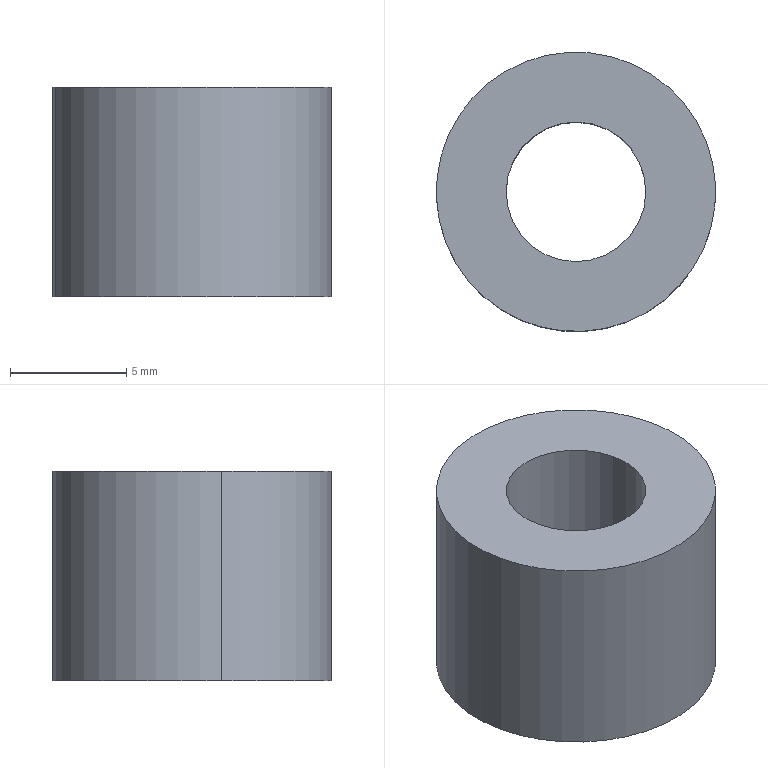Component | SolidWorks | ControlSleeve-1 | 1 solid | 6 faces | box 12 x 12 x 9 mm | volume 763 mm3 | cylinder 4 | plane 2 | commonest cylinder face diameters 6 x2 12 x2
build123d program:
from build123d import *

# Parameters (mm, degrees)
SKETCH1_R           = 6
SKETCH1_R_2         = 3
BOSS_EXTRUDE1_DEPTH = 9


with BuildPart() as part:
    # Sketch1 → Boss-Extrude1 (new body)
    with BuildSketch(Plane.XY):
        Circle(SKETCH1_R)
        Circle(SKETCH1_R_2, mode=Mode.SUBTRACT)
    extrude(amount=BOSS_EXTRUDE1_DEPTH)


solid = part.part

# Placed as in the assembly
solid = solid.moved(Location((3.727, 9.876, 358.846), (0, 0, 0)))
STEP:
#1=COLOUR_RGB('',0.7922,0.8196,0.9333);
#2=FILL_AREA_STYLE_COLOUR('',#1);
#3=FILL_AREA_STYLE('',(#2));
#4=SURFACE_STYLE_FILL_AREA(#3);
#5=SURFACE_SIDE_STYLE('',(#4));
#6=SURFACE_STYLE_USAGE(.BOTH.,#5);
#7=PRESENTATION_STYLE_ASSIGNMENT((#6));
#8=CARTESIAN_POINT('',(0.03129,0.3639,14.482));
#9=VERTEX_POINT('',#8);
#10=CARTESIAN_POINT('',(0.2622,0.4137,14.482));
#11=VERTEX_POINT('',#10);
#12=CARTESIAN_POINT('',(0.1467,0.3888,14.482));
#13=DIRECTION('',(0.,0.,1.));
#14=DIRECTION('',(0.9775,0.2111,0.));
#15=AXIS2_PLACEMENT_3D('',#12,#13,#14);
#16=CIRCLE('',#15,0.1181);
#17=EDGE_CURVE('',#9,#11,#16,.T.);
#18=ORIENTED_EDGE('',*,*,#17,.T.);
#19=CARTESIAN_POINT('',(0.2622,0.4137,14.128));
#20=VERTEX_POINT('',#19);
#21=CARTESIAN_POINT('',(0.2622,0.4137,14.482));
#22=DIRECTION('',(0.,0.,-1.));
#23=VECTOR('',#22,39.37);
#24=LINE('',#21,#23);
#25=EDGE_CURVE('',#11,#20,#24,.T.);
#26=ORIENTED_EDGE('',*,*,#25,.T.);
#27=CARTESIAN_POINT('',(0.03129,0.3639,14.128));
#28=VERTEX_POINT('',#27);
#29=CARTESIAN_POINT('',(0.1467,0.3888,14.128));
#30=DIRECTION('',(0.,0.,1.));
#31=DIRECTION('',(0.9775,0.2111,0.));
#32=AXIS2_PLACEMENT_3D('',#29,#30,#31);
#33=CIRCLE('',#32,0.1181);
#34=EDGE_CURVE('',#28,#20,#33,.T.);
#35=ORIENTED_EDGE('',*,*,#34,.F.);
#36=CARTESIAN_POINT('',(0.03129,0.3639,14.482));
#37=DIRECTION('',(0.,0.,-1.));
#38=VECTOR('',#37,39.37);
#39=LINE('',#36,#38);
#40=EDGE_CURVE('',#9,#28,#39,.T.);
#41=ORIENTED_EDGE('',*,*,#40,.F.);
#42=EDGE_LOOP('',(#18,#26,#35,#41));
#43=FACE_OUTER_BOUND('',#42,.T.);
#44=CARTESIAN_POINT('',(0.1467,0.3888,14.482));
#45=DIRECTION('',(0.,0.,-1.));
#46=DIRECTION('',(-0.9775,-0.2111,0.));
#47=AXIS2_PLACEMENT_3D('',#44,#45,#46);
#48=CYLINDRICAL_SURFACE('',#47,0.1181);
#49=ADVANCED_FACE('',(#43),#48,.F.);
#50=CARTESIAN_POINT('',(0.3776,0.4387,14.482));
#51=VERTEX_POINT('',#50);
#52=CARTESIAN_POINT('',(-0.08416,0.3389,14.482));
#53=VERTEX_POINT('',#52);
#54=CARTESIAN_POINT('',(0.1467,0.3888,14.482));
#55=DIRECTION('',(0.,0.,1.));
#56=DIRECTION('',(0.9775,0.2111,0.));
#57=AXIS2_PLACEMENT_3D('',#54,#55,#56);
#58=CIRCLE('',#57,0.2362);
#59=EDGE_CURVE('',#51,#53,#58,.T.);
#60=ORIENTED_EDGE('',*,*,#59,.F.);
#61=CARTESIAN_POINT('',(0.3776,0.4387,14.128));
#62=VERTEX_POINT('',#61);
#63=CARTESIAN_POINT('',(0.3776,0.4387,14.482));
#64=DIRECTION('',(0.,0.,-1.));
#65=VECTOR('',#64,39.37);
#66=LINE('',#63,#65);
#67=EDGE_CURVE('',#51,#62,#66,.T.);
#68=ORIENTED_EDGE('',*,*,#67,.T.);
#69=CARTESIAN_POINT('',(-0.08416,0.3389,14.128));
#70=VERTEX_POINT('',#69);
#71=CARTESIAN_POINT('',(0.1467,0.3888,14.128));
#72=DIRECTION('',(0.,0.,1.));
#73=DIRECTION('',(0.9775,0.2111,0.));
#74=AXIS2_PLACEMENT_3D('',#71,#72,#73);
#75=CIRCLE('',#74,0.2362);
#76=EDGE_CURVE('',#62,#70,#75,.T.);
#77=ORIENTED_EDGE('',*,*,#76,.T.);
#78=CARTESIAN_POINT('',(-0.08416,0.3389,14.482));
#79=DIRECTION('',(0.,0.,-1.));
#80=VECTOR('',#79,39.37);
#81=LINE('',#78,#80);
#82=EDGE_CURVE('',#53,#70,#81,.T.);
#83=ORIENTED_EDGE('',*,*,#82,.F.);
#84=EDGE_LOOP('',(#60,#68,#77,#83));
#85=FACE_OUTER_BOUND('',#84,.T.);
#86=CARTESIAN_POINT('',(0.1467,0.3888,14.482));
#87=DIRECTION('',(0.,0.,-1.));
#88=DIRECTION('',(-0.9775,-0.2111,0.));
#89=AXIS2_PLACEMENT_3D('',#86,#87,#88);
#90=CYLINDRICAL_SURFACE('',#89,0.2362);
#91=ADVANCED_FACE('',(#85),#90,.T.);
#92=CARTESIAN_POINT('',(0.1467,0.3888,14.482));
#93=DIRECTION('',(0.,0.,1.));
#94=DIRECTION('',(0.9775,0.2111,0.));
#95=AXIS2_PLACEMENT_3D('',#92,#93,#94);
#96=CIRCLE('',#95,0.2362);
#97=EDGE_CURVE('',#53,#51,#96,.T.);
#98=ORIENTED_EDGE('',*,*,#97,.T.);
#99=ORIENTED_EDGE('',*,*,#59,.T.);
#100=EDGE_LOOP('',(#98,#99));
#101=FACE_OUTER_BOUND('',#100,.T.);
#102=ORIENTED_EDGE('',*,*,#17,.F.);
#103=CARTESIAN_POINT('',(0.1467,0.3888,14.482));
#104=DIRECTION('',(0.,0.,1.));
#105=DIRECTION('',(0.9775,0.2111,0.));
#106=AXIS2_PLACEMENT_3D('',#103,#104,#105);
#107=CIRCLE('',#106,0.1181);
#108=EDGE_CURVE('',#11,#9,#107,.T.);
#109=ORIENTED_EDGE('',*,*,#108,.F.);
#110=EDGE_LOOP('',(#102,#109));
#111=FACE_BOUND('',#110,.T.);
#112=CARTESIAN_POINT('',(0.1467,0.3888,14.482));
#113=DIRECTION('',(0.,0.,1.));
#114=DIRECTION('',(0.9775,0.2111,0.));
#115=AXIS2_PLACEMENT_3D('',#112,#113,#114);
#116=PLANE('',#115);
#117=ADVANCED_FACE('',(#101,#111),#116,.T.);
#118=CARTESIAN_POINT('',(0.1467,0.3888,14.128));
#119=DIRECTION('',(0.,0.,1.));
#120=DIRECTION('',(0.9775,0.2111,0.));
#121=AXIS2_PLACEMENT_3D('',#118,#119,#120);
#122=CIRCLE('',#121,0.2362);
#123=EDGE_CURVE('',#70,#62,#122,.T.);
#124=ORIENTED_EDGE('',*,*,#123,.F.);
#125=ORIENTED_EDGE('',*,*,#76,.F.);
#126=EDGE_LOOP('',(#124,#125));
#127=FACE_OUTER_BOUND('',#126,.T.);
#128=ORIENTED_EDGE('',*,*,#34,.T.);
#129=CARTESIAN_POINT('',(0.1467,0.3888,14.128));
#130=DIRECTION('',(0.,0.,1.));
#131=DIRECTION('',(0.9775,0.2111,0.));
#132=AXIS2_PLACEMENT_3D('',#129,#130,#131);
#133=CIRCLE('',#132,0.1181);
#134=EDGE_CURVE('',#20,#28,#133,.T.);
#135=ORIENTED_EDGE('',*,*,#134,.T.);
#136=EDGE_LOOP('',(#128,#135));
#137=FACE_BOUND('',#136,.T.);
#138=CARTESIAN_POINT('',(0.1467,0.3888,14.128));
#139=DIRECTION('',(0.,0.,1.));
#140=DIRECTION('',(0.9775,0.2111,0.));
#141=AXIS2_PLACEMENT_3D('',#138,#139,#140);
#142=PLANE('',#141);
#143=ADVANCED_FACE('',(#127,#137),#142,.F.);
#144=ORIENTED_EDGE('',*,*,#67,.F.);
#145=ORIENTED_EDGE('',*,*,#97,.F.);
#146=ORIENTED_EDGE('',*,*,#82,.T.);
#147=ORIENTED_EDGE('',*,*,#123,.T.);
#148=EDGE_LOOP('',(#144,#145,#146,#147));
#149=FACE_OUTER_BOUND('',#148,.T.);
#150=CARTESIAN_POINT('',(0.1467,0.3888,14.482));
#151=DIRECTION('',(0.,0.,-1.));
#152=DIRECTION('',(-0.9775,-0.2111,0.));
#153=AXIS2_PLACEMENT_3D('',#150,#151,#152);
#154=CYLINDRICAL_SURFACE('',#153,0.2362);
#155=ADVANCED_FACE('',(#149),#154,.T.);
#156=ORIENTED_EDGE('',*,*,#25,.F.);
#157=ORIENTED_EDGE('',*,*,#108,.T.);
#158=ORIENTED_EDGE('',*,*,#40,.T.);
#159=ORIENTED_EDGE('',*,*,#134,.F.);
#160=EDGE_LOOP('',(#156,#157,#158,#159));
#161=FACE_OUTER_BOUND('',#160,.T.);
#162=CARTESIAN_POINT('',(0.1467,0.3888,14.482));
#163=DIRECTION('',(0.,0.,-1.));
#164=DIRECTION('',(-0.9775,-0.2111,0.));
#165=AXIS2_PLACEMENT_3D('',#162,#163,#164);
#166=CYLINDRICAL_SURFACE('',#165,0.1181);
#167=ADVANCED_FACE('',(#161),#166,.F.);
#168=CLOSED_SHELL('',(#49,#91,#117,#143,#155,#167));
#169=MANIFOLD_SOLID_BREP('',#168);
#170=STYLED_ITEM('',(#7),#169);
#171=PRESENTATION_LAYER_ASSIGNMENT('','',(#170));
#172=(LENGTH_UNIT()NAMED_UNIT(*)SI_UNIT($,.METRE.));
#173=LENGTH_MEASURE_WITH_UNIT(LENGTH_MEASURE(0.0254),#172);
#174=DIMENSIONAL_EXPONENTS(1.,0.,0.,0.,0.,0.,0.);
#175=(CONVERSION_BASED_UNIT('',#173)LENGTH_UNIT()NAMED_UNIT(#174));
#176=UNCERTAINTY_MEASURE_WITH_UNIT(LENGTH_MEASURE(0.00001),#175,'','');
#177=(NAMED_UNIT(*)PLANE_ANGLE_UNIT()SI_UNIT($,.RADIAN.));
#178=(NAMED_UNIT(*)SI_UNIT($,.STERADIAN.)SOLID_ANGLE_UNIT());
#179=(GEOMETRIC_REPRESENTATION_CONTEXT(3)GLOBAL_UNCERTAINTY_ASSIGNED_CONTEXT((#176))GLOBAL_UNIT_ASSIGNED_CONTEXT((#175,#177,#178))REPRESENTATION_CONTEXT('',''));
#180=MECHANICAL_DESIGN_GEOMETRIC_PRESENTATION_REPRESENTATION('',(#170),#179);
#181=CARTESIAN_POINT('',(0.,0.,0.));
#182=DIRECTION('',(0.,0.,1.));
#183=DIRECTION('',(1.,0.,0.));
#184=AXIS2_PLACEMENT_3D('',#181,#182,#183);
#185=(LENGTH_UNIT()NAMED_UNIT(*)SI_UNIT($,.METRE.));
#186=LENGTH_MEASURE_WITH_UNIT(LENGTH_MEASURE(0.0254),#185);
#187=DIMENSIONAL_EXPONENTS(1.,0.,0.,0.,0.,0.,0.);
#188=(CONVERSION_BASED_UNIT('',#186)LENGTH_UNIT()NAMED_UNIT(#187));
#189=UNCERTAINTY_MEASURE_WITH_UNIT(LENGTH_MEASURE(0.00001),#188,'','');
#190=(NAMED_UNIT(*)PLANE_ANGLE_UNIT()SI_UNIT($,.RADIAN.));
#191=(NAMED_UNIT(*)SI_UNIT($,.STERADIAN.)SOLID_ANGLE_UNIT());
#192=(GEOMETRIC_REPRESENTATION_CONTEXT(3)GLOBAL_UNCERTAINTY_ASSIGNED_CONTEXT((#189))GLOBAL_UNIT_ASSIGNED_CONTEXT((#188,#190,#191))REPRESENTATION_CONTEXT('',''));
#193=ADVANCED_BREP_SHAPE_REPRESENTATION('',(#169,#184),#192);